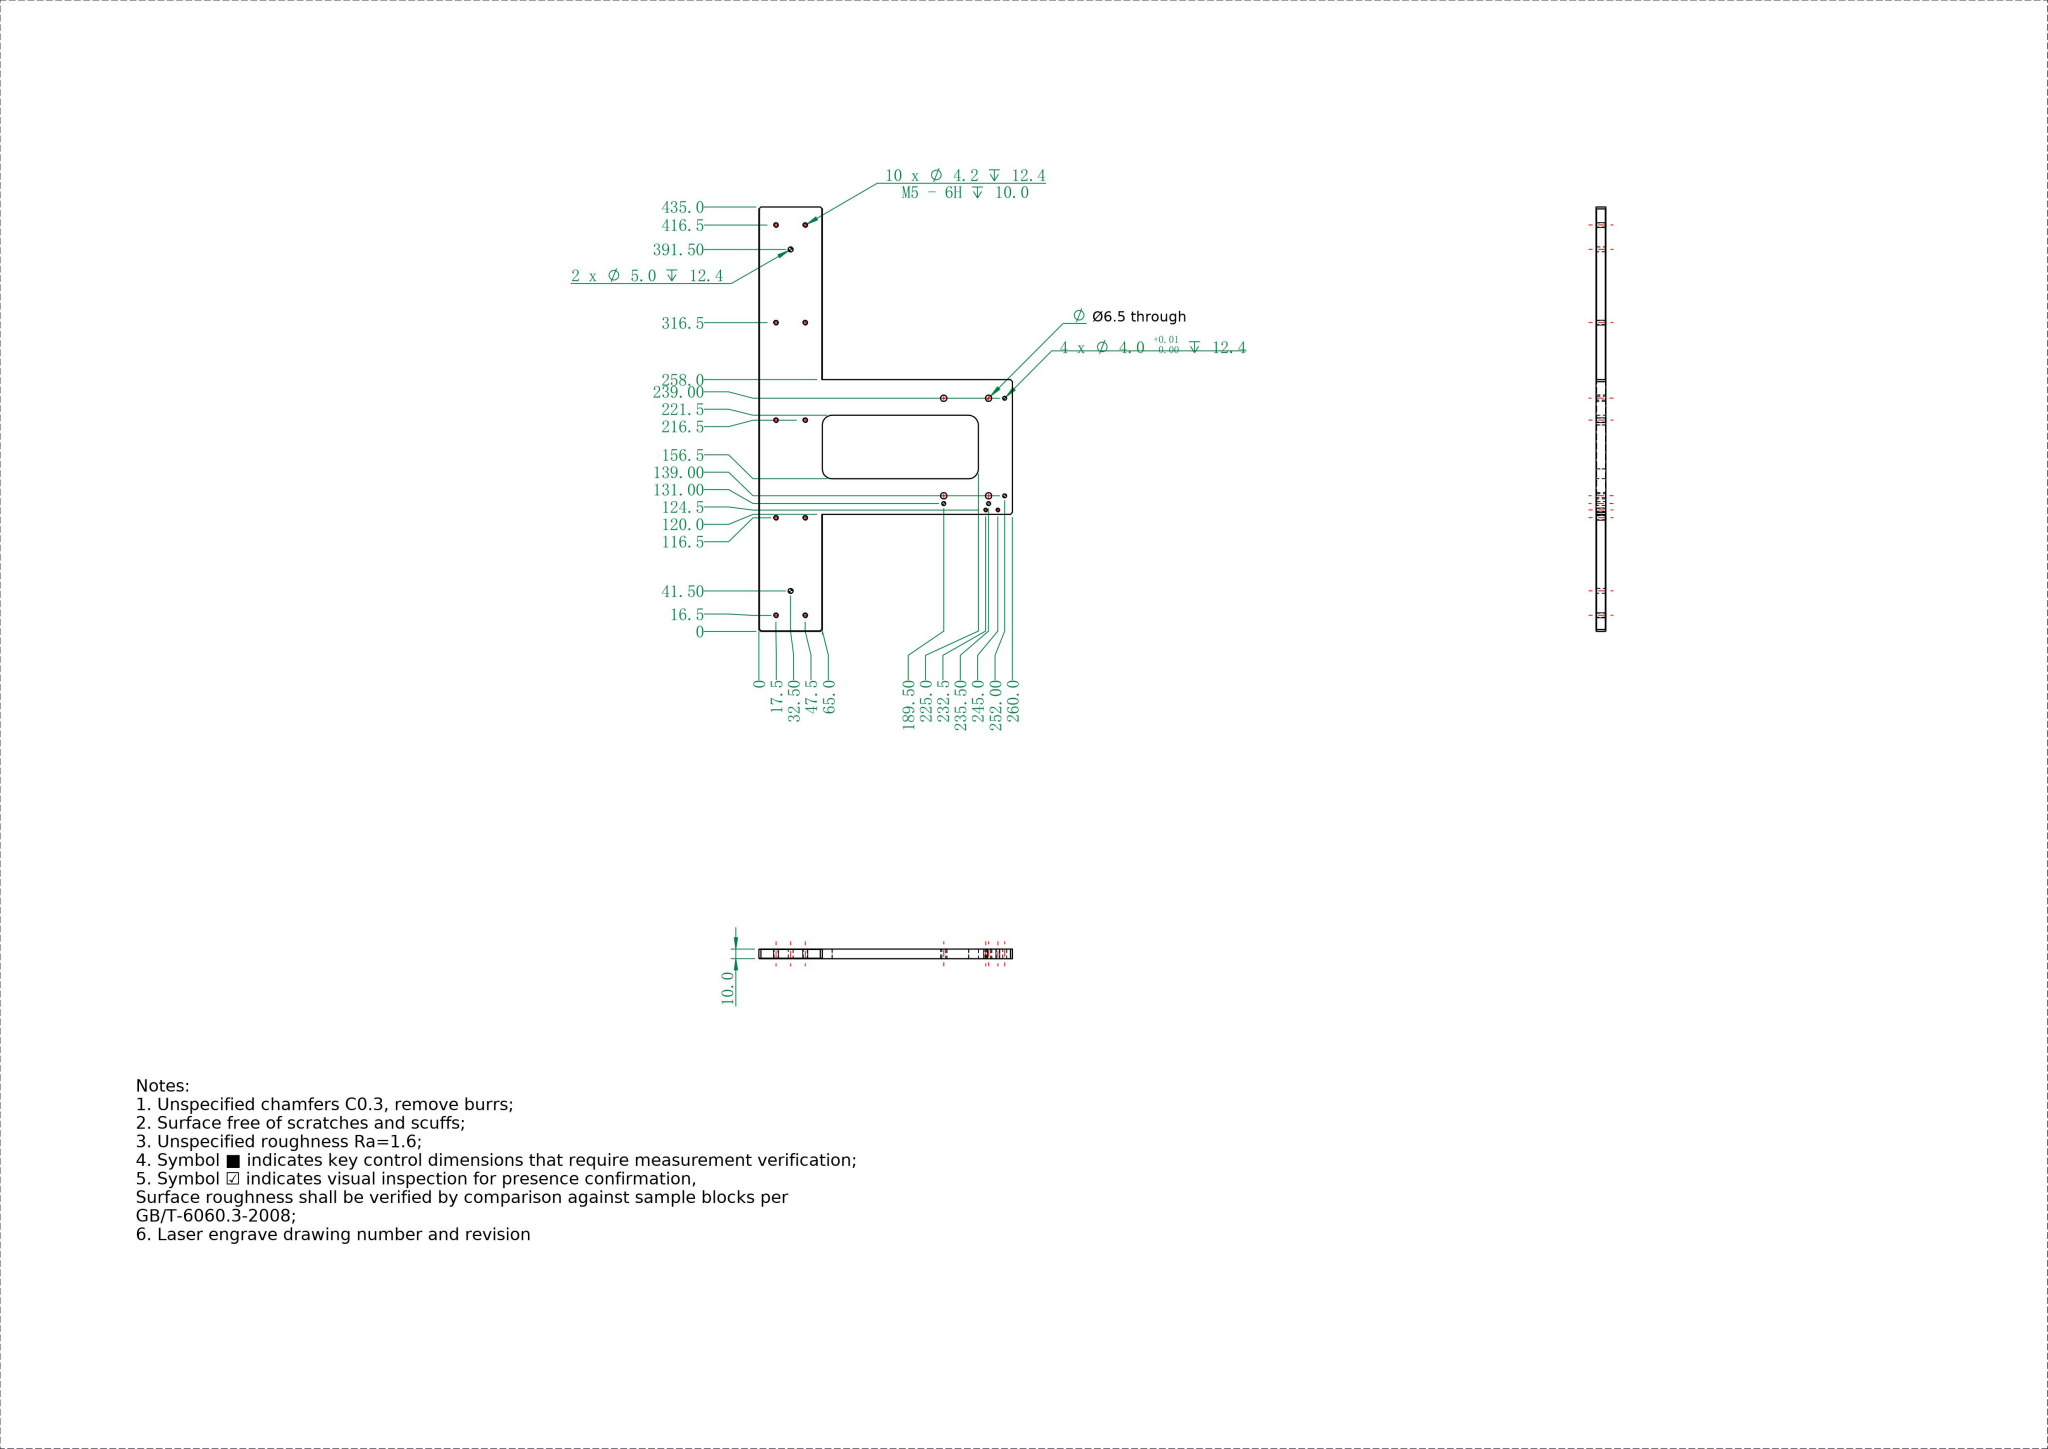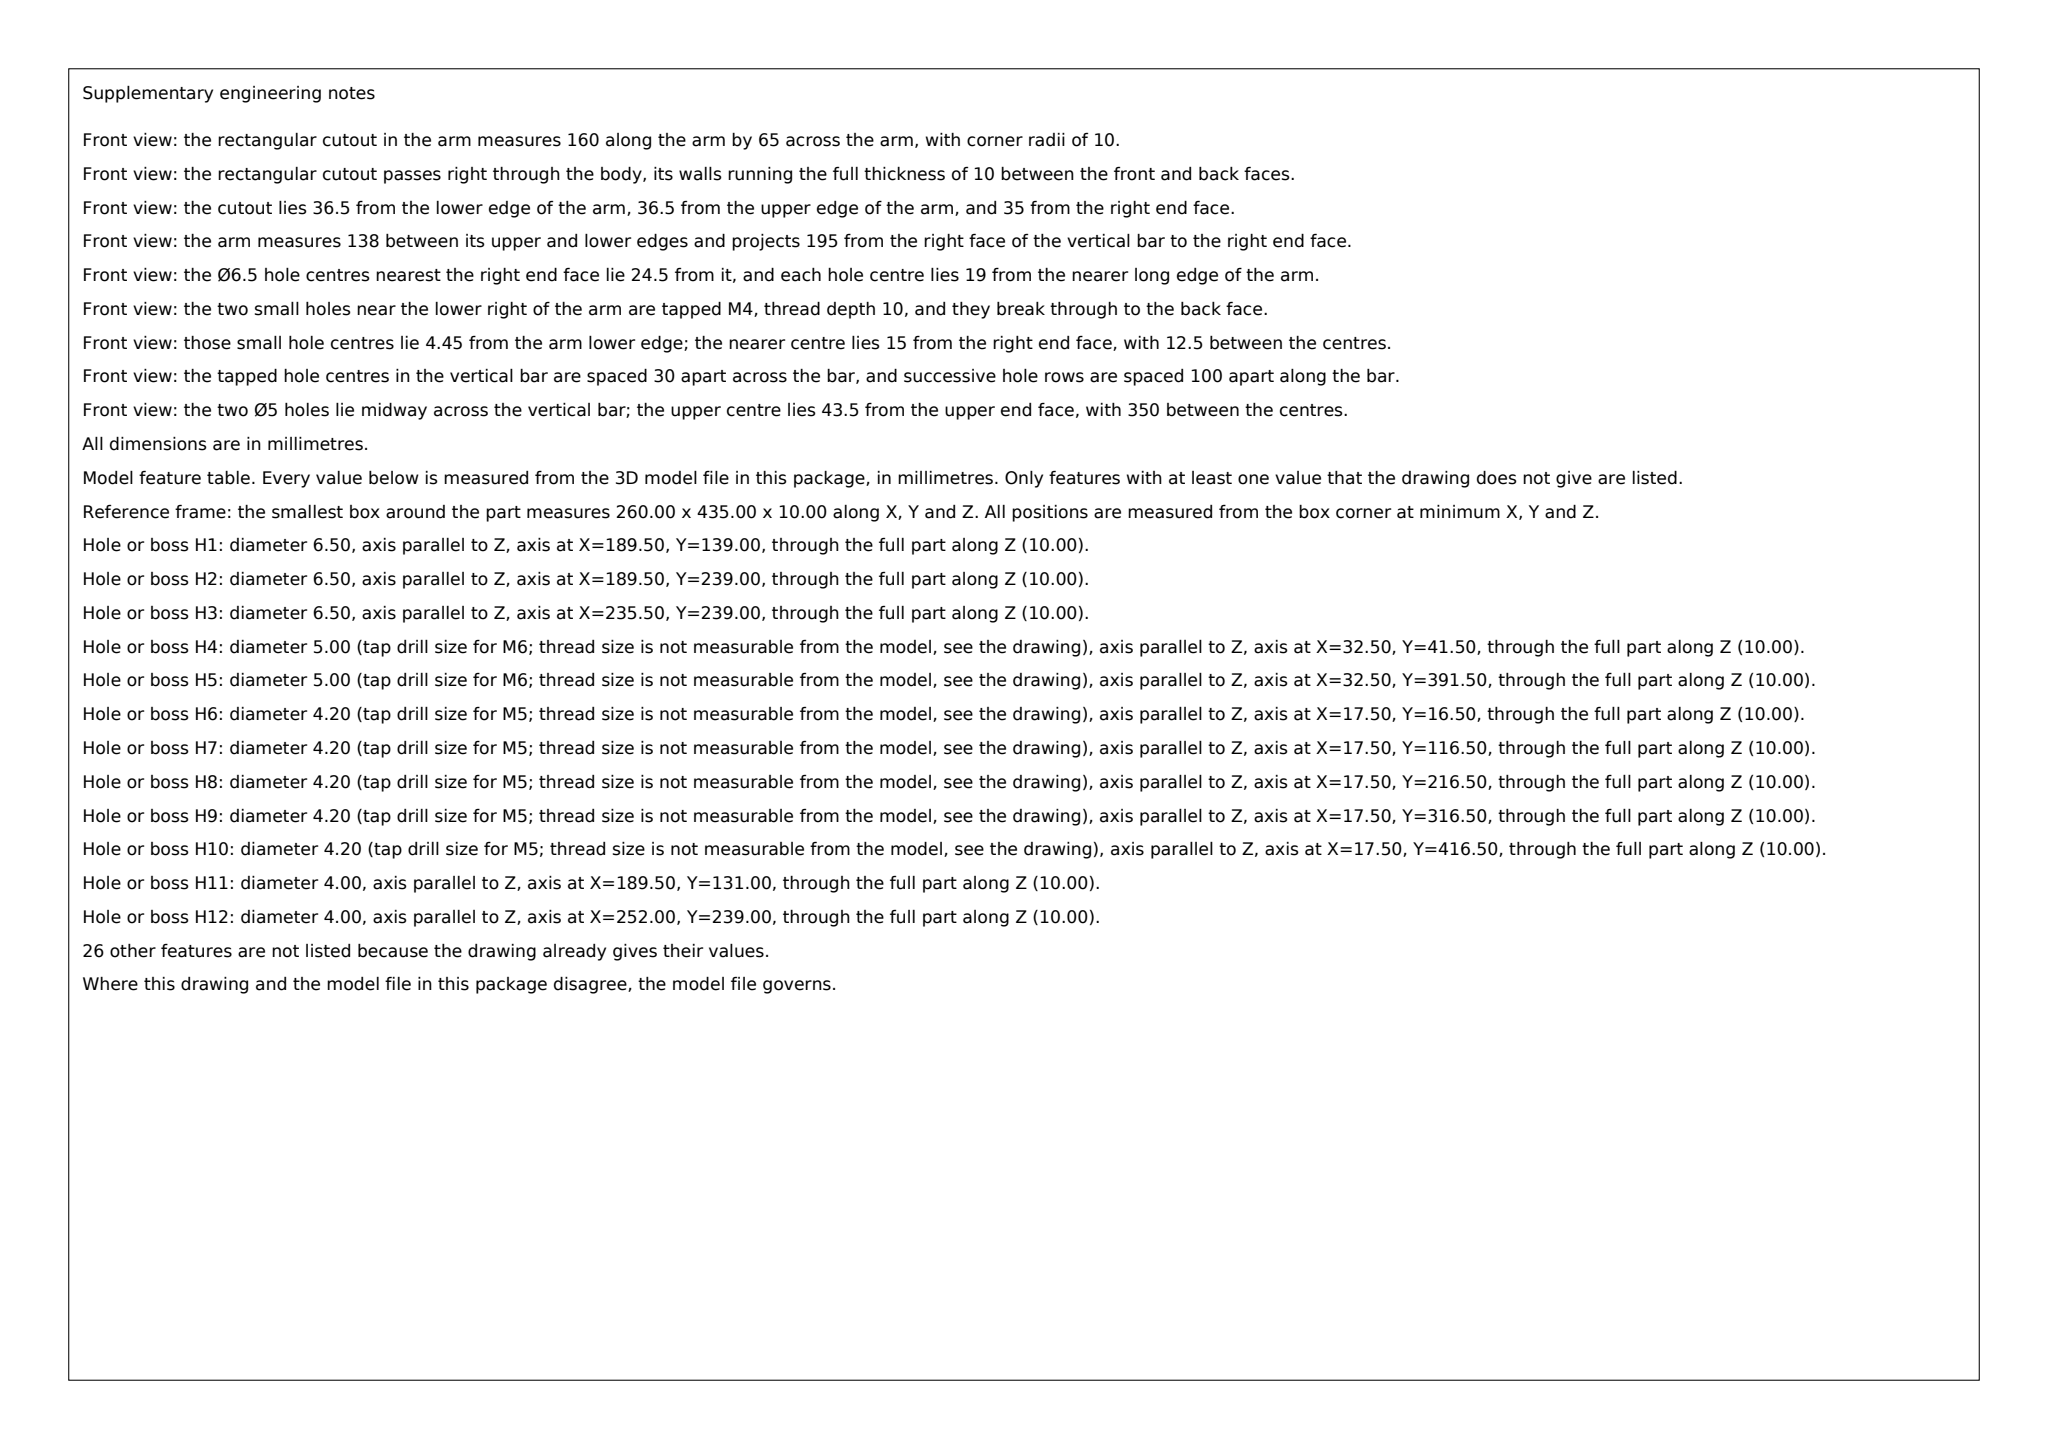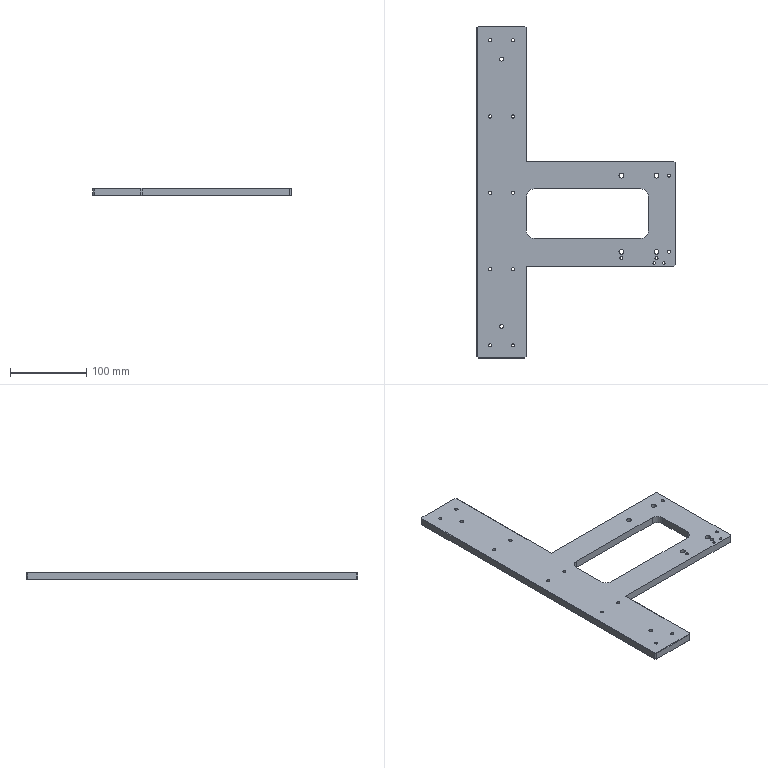Part | SolidWorks | mm | 1 solid | 80 faces | box 260 x 435 x 10 mm | volume 444612 mm3 | cylinder 48 | plane 32 | commonest cylinder face diameters 4.2 x20 4 x8 6.5 x8 3.3 x4 5 x4 20 x4